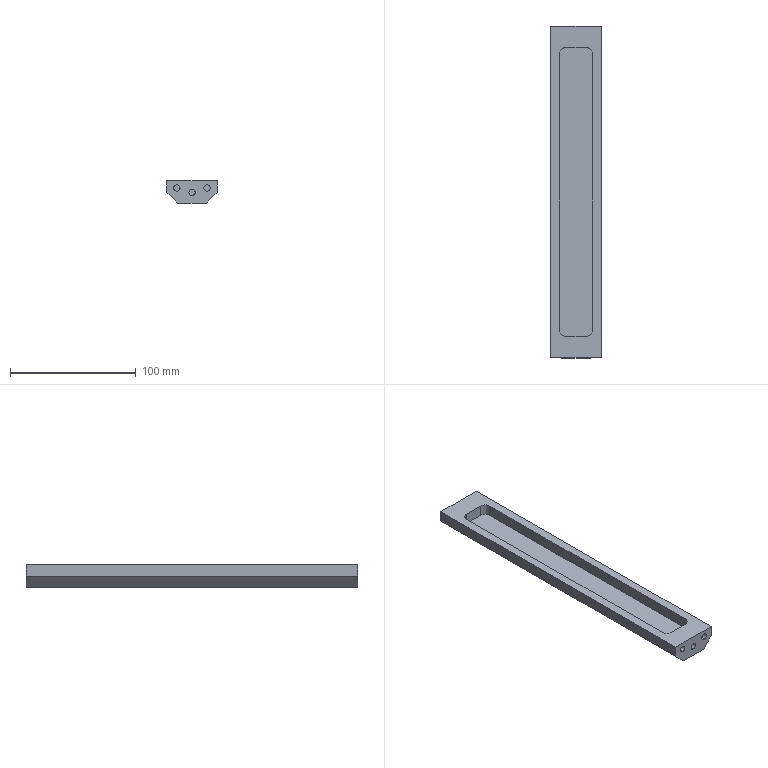CAM job | Mastercam | mm | 14 operations | part box 40 x 264 x 17.69
1. Facing | 24 - 100 平铣刀
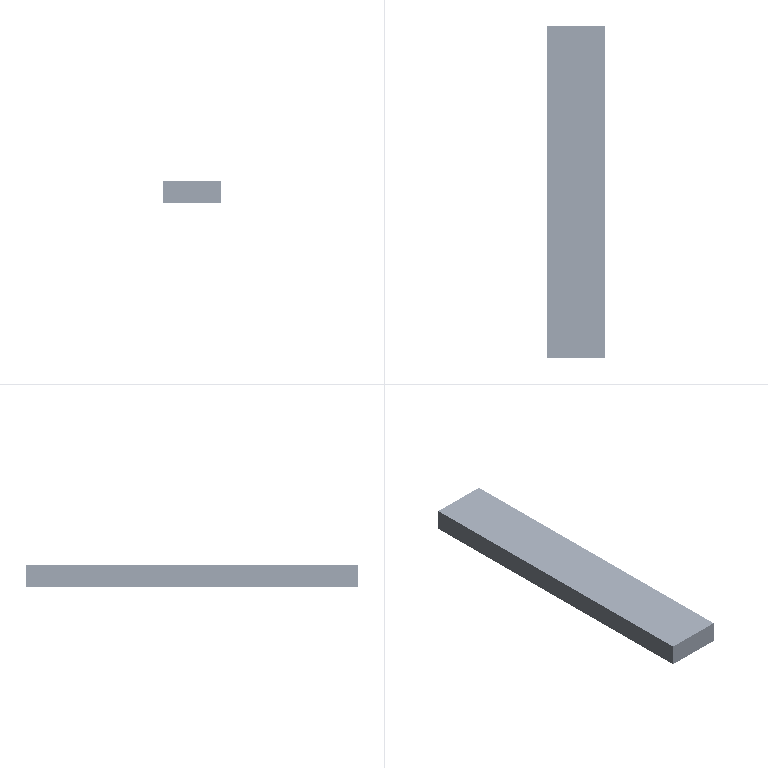2. Contour (Ramp) | 16 - 16 平铣刀
3. Contour (Ramp) | 16 - 16 平铣刀
4. Contour (2D) | 10 - 10 平铣刀
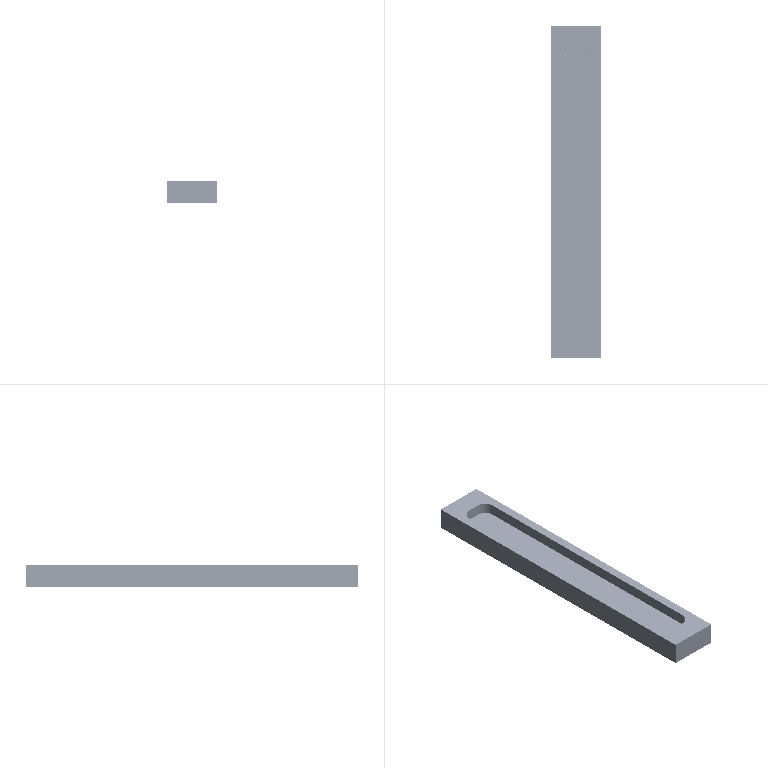5. Contour (Remachining) | 10 - 10 平铣刀
6. 2D High Speed (2D Area Mill) | 10 - 10 平铣刀
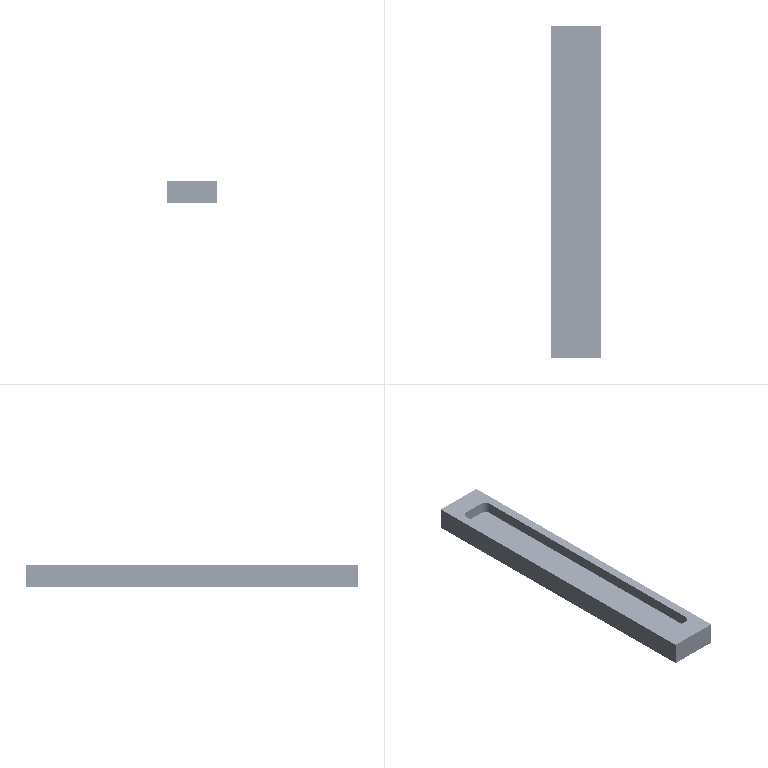7. Contour (2D) | 10 - 10 平铣刀
8. Contour (2D chamfer) | 7 - 4 倒角刀
9. Facing | 24 - 100 平铣刀
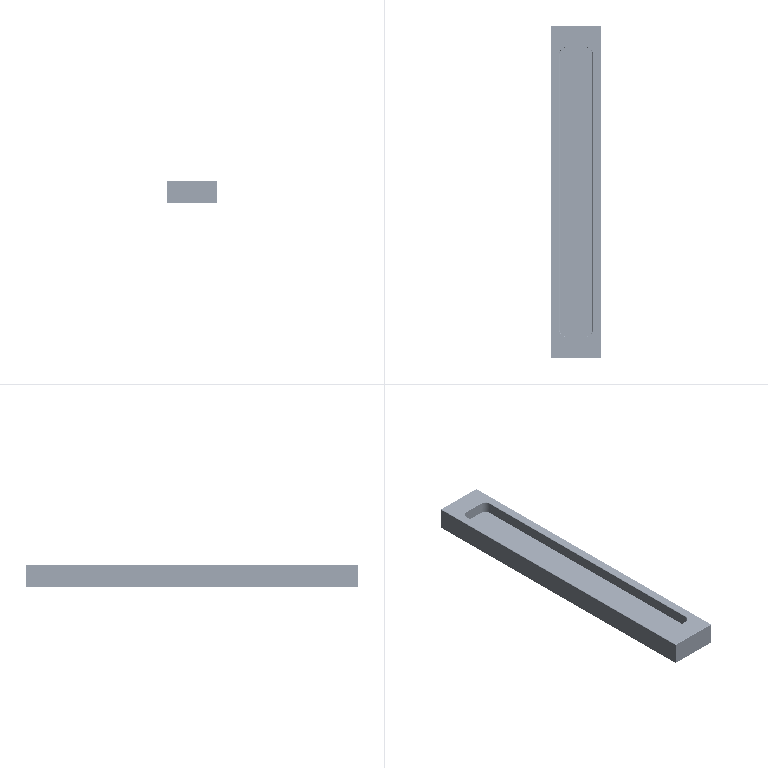10. Surface Finish Flowline | 11 - 10 圆鼻铣刀
11. Deburr 5-axis | 5 - 4 球刀/圆鼻铣刀
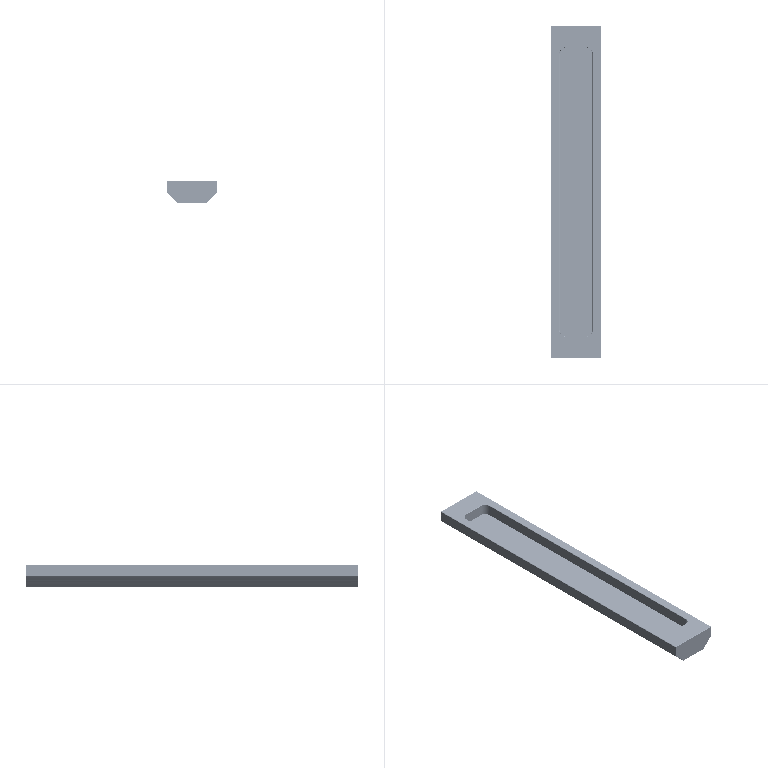12. Drill/Counterbore | 7 - 4 倒角刀
13. Peck Drill | 1 - 5.1 钻头
14. Contour (2D chamfer) | 7 - 4 倒角刀